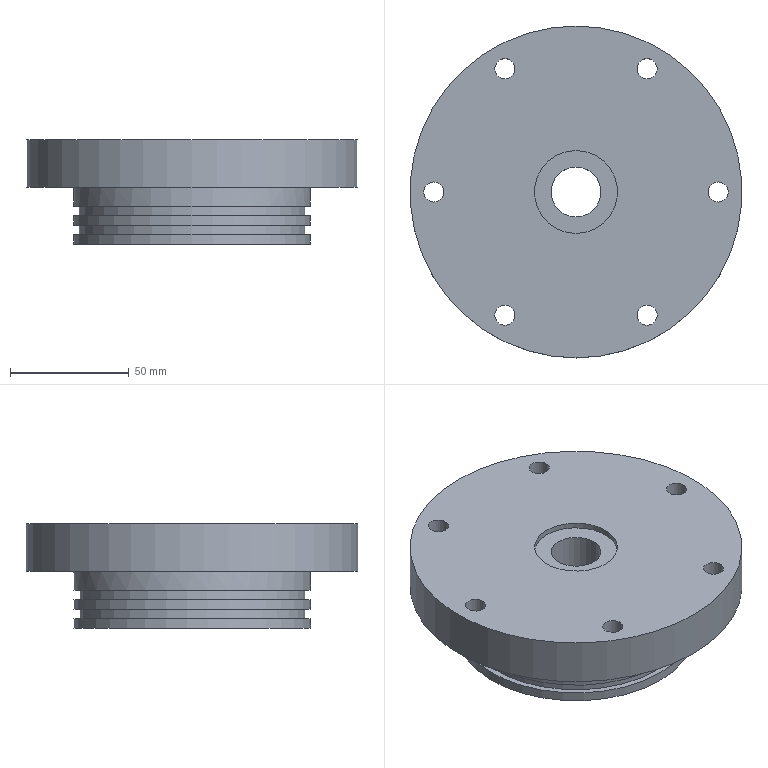Component | NX | CYLINDER_HEAD | 1 solid | 26 faces | volume 451793 mm3 | cylinder 16 | plane 10 | commonest cylinder face diameters 8.5 x6 100 x3 95.2 x2 140 x1 35 x1 50 x1 40 x1 21 x1